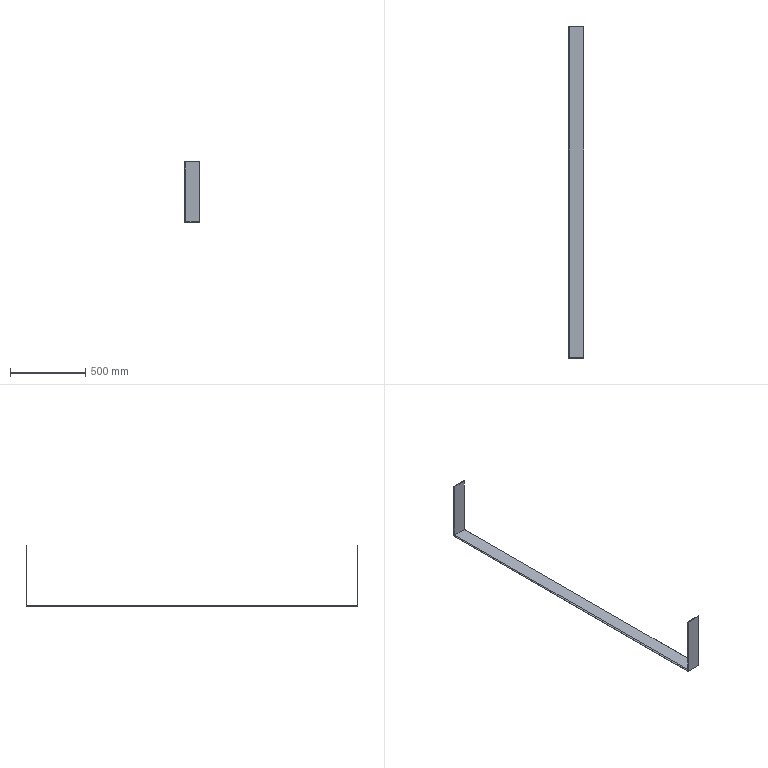Component | NX | FACA | 1 solid | 13 faces | box 100 x 2210 x 400 mm | volume 1452075 mm3 | plane 13
STEP:
#1=CARTESIAN_POINT('',(0.,0.,0.));
#2=DIRECTION('',(0.,0.,1.));
#3=DIRECTION('',(1.,0.,0.));
#4=AXIS2_PLACEMENT_3D('',#1,#2,#3);
#5=CARTESIAN_POINT('',(-710.,770.167,480.));
#6=VERTEX_POINT('',#5);
#7=CARTESIAN_POINT('',(-710.,770.167,80.));
#8=VERTEX_POINT('',#7);
#9=CARTESIAN_POINT('',(-710.,770.167,480.));
#10=DIRECTION('',(0.,0.,-1.));
#11=VECTOR('',#10,1.);
#12=LINE('',#9,#11);
#13=CARTESIAN_POINT('',(-810.,770.167,480.));
#14=DIRECTION('',(0.,-1.,0.));
#15=DIRECTION('',(0.,0.,1.));
#16=AXIS2_PLACEMENT_3D('',#13,#14,#15);
#17=PLANE('',#16);
#18=CARTESIAN_POINT('',(0.,-100.));
#19=DIRECTION('',(-1.,0.));
#20=VECTOR('',#19,1.);
#21=LINE('',#18,#20);
#22=(GEOMETRIC_REPRESENTATION_CONTEXT(2)PARAMETRIC_REPRESENTATION_CONTEXT()REPRESENTATION_CONTEXT('',''));
#23=DEFINITIONAL_REPRESENTATION('',(#21),#22);
#24=PCURVE('',#17,#23);
#25=CARTESIAN_POINT('',(-710.,770.167,80.));
#26=DIRECTION('',(-1.,0.,0.));
#27=DIRECTION('',(0.,0.,-1.));
#28=AXIS2_PLACEMENT_3D('',#25,#26,#27);
#29=PLANE('',#28);
#30=CARTESIAN_POINT('',(-400.,0.));
#31=DIRECTION('',(1.,0.));
#32=VECTOR('',#31,1.);
#33=LINE('',#30,#32);
#34=(GEOMETRIC_REPRESENTATION_CONTEXT(2)PARAMETRIC_REPRESENTATION_CONTEXT()REPRESENTATION_CONTEXT('',''));
#35=DEFINITIONAL_REPRESENTATION('',(#33),#34);
#36=PCURVE('',#29,#35);
#37=SURFACE_CURVE('',#12,(#24,#36),.PCURVE_S1.);
#38=EDGE_CURVE('',#6,#8,#37,.T.);
#39=ORIENTED_EDGE('',*,*,#38,.T.);
#40=CARTESIAN_POINT('',(-810.,770.167,80.));
#41=VERTEX_POINT('',#40);
#42=CARTESIAN_POINT('',(-810.,770.167,80.));
#43=DIRECTION('',(1.,0.,0.));
#44=VECTOR('',#43,1.);
#45=LINE('',#42,#44);
#46=CARTESIAN_POINT('',(-400.,0.));
#47=DIRECTION('',(0.,-1.));
#48=VECTOR('',#47,1.);
#49=LINE('',#46,#48);
#50=(GEOMETRIC_REPRESENTATION_CONTEXT(2)PARAMETRIC_REPRESENTATION_CONTEXT()REPRESENTATION_CONTEXT('',''));
#51=DEFINITIONAL_REPRESENTATION('',(#49),#50);
#52=PCURVE('',#17,#51);
#53=CARTESIAN_POINT('',(-810.,770.167,80.));
#54=DIRECTION('',(0.,0.,1.));
#55=DIRECTION('',(-1.,0.,0.));
#56=AXIS2_PLACEMENT_3D('',#53,#54,#55);
#57=PLANE('',#56);
#58=CARTESIAN_POINT('',(0.,0.));
#59=DIRECTION('',(-1.,0.));
#60=VECTOR('',#59,1.);
#61=LINE('',#58,#60);
#62=(GEOMETRIC_REPRESENTATION_CONTEXT(2)PARAMETRIC_REPRESENTATION_CONTEXT()REPRESENTATION_CONTEXT('',''));
#63=DEFINITIONAL_REPRESENTATION('',(#61),#62);
#64=PCURVE('',#57,#63);
#65=SURFACE_CURVE('',#45,(#52,#64),.PCURVE_S1.);
#66=EDGE_CURVE('',#41,#8,#65,.T.);
#67=ORIENTED_EDGE('',*,*,#66,.F.);
#68=CARTESIAN_POINT('',(-810.,770.167,480.));
#69=VERTEX_POINT('',#68);
#70=CARTESIAN_POINT('',(-810.,770.167,480.));
#71=DIRECTION('',(0.,0.,-1.));
#72=VECTOR('',#71,1.);
#73=LINE('',#70,#72);
#74=CARTESIAN_POINT('',(0.,0.));
#75=DIRECTION('',(-1.,0.));
#76=VECTOR('',#75,1.);
#77=LINE('',#74,#76);
#78=(GEOMETRIC_REPRESENTATION_CONTEXT(2)PARAMETRIC_REPRESENTATION_CONTEXT()REPRESENTATION_CONTEXT('',''));
#79=DEFINITIONAL_REPRESENTATION('',(#77),#78);
#80=PCURVE('',#17,#79);
#81=CARTESIAN_POINT('',(-810.,770.167,80.));
#82=DIRECTION('',(-1.,0.,0.));
#83=DIRECTION('',(0.,0.,-1.));
#84=AXIS2_PLACEMENT_3D('',#81,#82,#83);
#85=PLANE('',#84);
#86=CARTESIAN_POINT('',(-400.,0.));
#87=DIRECTION('',(1.,0.));
#88=VECTOR('',#87,1.);
#89=LINE('',#86,#88);
#90=(GEOMETRIC_REPRESENTATION_CONTEXT(2)PARAMETRIC_REPRESENTATION_CONTEXT()REPRESENTATION_CONTEXT('',''));
#91=DEFINITIONAL_REPRESENTATION('',(#89),#90);
#92=PCURVE('',#85,#91);
#93=SURFACE_CURVE('',#73,(#80,#92),.PCURVE_S1.);
#94=EDGE_CURVE('',#69,#41,#93,.T.);
#95=ORIENTED_EDGE('',*,*,#94,.F.);
#96=CARTESIAN_POINT('',(-810.,770.167,480.));
#97=DIRECTION('',(1.,0.,0.));
#98=VECTOR('',#97,1.);
#99=LINE('',#96,#98);
#100=CARTESIAN_POINT('',(0.,0.));
#101=DIRECTION('',(0.,-1.));
#102=VECTOR('',#101,1.);
#103=LINE('',#100,#102);
#104=(GEOMETRIC_REPRESENTATION_CONTEXT(2)PARAMETRIC_REPRESENTATION_CONTEXT()REPRESENTATION_CONTEXT('',''));
#105=DEFINITIONAL_REPRESENTATION('',(#103),#104);
#106=PCURVE('',#17,#105);
#107=CARTESIAN_POINT('',(-810.,765.167,480.));
#108=DIRECTION('',(0.,0.,-1.));
#109=DIRECTION('',(1.,0.,0.));
#110=AXIS2_PLACEMENT_3D('',#107,#108,#109);
#111=PLANE('',#110);
#112=CARTESIAN_POINT('',(0.,-5.));
#113=DIRECTION('',(1.,0.));
#114=VECTOR('',#113,1.);
#115=LINE('',#112,#114);
#116=(GEOMETRIC_REPRESENTATION_CONTEXT(2)PARAMETRIC_REPRESENTATION_CONTEXT()REPRESENTATION_CONTEXT('',''));
#117=DEFINITIONAL_REPRESENTATION('',(#115),#116);
#118=PCURVE('',#111,#117);
#119=SURFACE_CURVE('',#99,(#106,#118),.PCURVE_S1.);
#120=EDGE_CURVE('',#69,#6,#119,.T.);
#121=ORIENTED_EDGE('',*,*,#120,.T.);
#122=EDGE_LOOP('',(#39,#67,#95,#121));
#123=FACE_BOUND('',#122,.T.);
#124=ADVANCED_FACE('',(#123),#17,.F.);
#125=CARTESIAN_POINT('',(-710.,-1439.833,80.));
#126=VERTEX_POINT('',#125);
#127=CARTESIAN_POINT('',(-710.,770.167,80.));
#128=DIRECTION('',(0.,-1.,0.));
#129=VECTOR('',#128,1.);
#130=LINE('',#127,#129);
#131=CARTESIAN_POINT('',(-100.,0.));
#132=DIRECTION('',(0.,1.));
#133=VECTOR('',#132,1.);
#134=LINE('',#131,#133);
#135=(GEOMETRIC_REPRESENTATION_CONTEXT(2)PARAMETRIC_REPRESENTATION_CONTEXT()REPRESENTATION_CONTEXT('',''));
#136=DEFINITIONAL_REPRESENTATION('',(#134),#135);
#137=PCURVE('',#57,#136);
#138=CARTESIAN_POINT('',(0.,0.));
#139=DIRECTION('',(0.,1.));
#140=VECTOR('',#139,1.);
#141=LINE('',#138,#140);
#142=(GEOMETRIC_REPRESENTATION_CONTEXT(2)PARAMETRIC_REPRESENTATION_CONTEXT()REPRESENTATION_CONTEXT('',''));
#143=DEFINITIONAL_REPRESENTATION('',(#141),#142);
#144=PCURVE('',#29,#143);
#145=SURFACE_CURVE('',#130,(#137,#144),.PCURVE_S1.);
#146=EDGE_CURVE('',#8,#126,#145,.T.);
#147=ORIENTED_EDGE('',*,*,#146,.T.);
#148=CARTESIAN_POINT('',(-810.,-1439.833,80.));
#149=VERTEX_POINT('',#148);
#150=CARTESIAN_POINT('',(-810.,-1439.833,80.));
#151=DIRECTION('',(1.,0.,0.));
#152=VECTOR('',#151,1.);
#153=LINE('',#150,#152);
#154=CARTESIAN_POINT('',(0.,2210.));
#155=DIRECTION('',(-1.,0.));
#156=VECTOR('',#155,1.);
#157=LINE('',#154,#156);
#158=(GEOMETRIC_REPRESENTATION_CONTEXT(2)PARAMETRIC_REPRESENTATION_CONTEXT()REPRESENTATION_CONTEXT('',''));
#159=DEFINITIONAL_REPRESENTATION('',(#157),#158);
#160=PCURVE('',#57,#159);
#161=CARTESIAN_POINT('',(-810.,-1439.833,80.));
#162=DIRECTION('',(0.,1.,0.));
#163=DIRECTION('',(0.,0.,-1.));
#164=AXIS2_PLACEMENT_3D('',#161,#162,#163);
#165=PLANE('',#164);
#166=CARTESIAN_POINT('',(0.,0.));
#167=DIRECTION('',(0.,-1.));
#168=VECTOR('',#167,1.);
#169=LINE('',#166,#168);
#170=(GEOMETRIC_REPRESENTATION_CONTEXT(2)PARAMETRIC_REPRESENTATION_CONTEXT()REPRESENTATION_CONTEXT('',''));
#171=DEFINITIONAL_REPRESENTATION('',(#169),#170);
#172=PCURVE('',#165,#171);
#173=SURFACE_CURVE('',#153,(#160,#172),.PCURVE_S1.);
#174=EDGE_CURVE('',#149,#126,#173,.T.);
#175=ORIENTED_EDGE('',*,*,#174,.F.);
#176=CARTESIAN_POINT('',(-810.,770.167,80.));
#177=DIRECTION('',(0.,-1.,0.));
#178=VECTOR('',#177,1.);
#179=LINE('',#176,#178);
#180=CARTESIAN_POINT('',(0.,0.));
#181=DIRECTION('',(0.,1.));
#182=VECTOR('',#181,1.);
#183=LINE('',#180,#182);
#184=(GEOMETRIC_REPRESENTATION_CONTEXT(2)PARAMETRIC_REPRESENTATION_CONTEXT()REPRESENTATION_CONTEXT('',''));
#185=DEFINITIONAL_REPRESENTATION('',(#183),#184);
#186=PCURVE('',#57,#185);
#187=CARTESIAN_POINT('',(0.,0.));
#188=DIRECTION('',(0.,1.));
#189=VECTOR('',#188,1.);
#190=LINE('',#187,#189);
#191=(GEOMETRIC_REPRESENTATION_CONTEXT(2)PARAMETRIC_REPRESENTATION_CONTEXT()REPRESENTATION_CONTEXT('',''));
#192=DEFINITIONAL_REPRESENTATION('',(#190),#191);
#193=PCURVE('',#85,#192);
#194=SURFACE_CURVE('',#179,(#186,#193),.PCURVE_S1.);
#195=EDGE_CURVE('',#41,#149,#194,.T.);
#196=ORIENTED_EDGE('',*,*,#195,.F.);
#197=ORIENTED_EDGE('',*,*,#66,.T.);
#198=EDGE_LOOP('',(#147,#175,#196,#197));
#199=FACE_BOUND('',#198,.T.);
#200=ADVANCED_FACE('',(#199),#57,.F.);
#201=CARTESIAN_POINT('',(-710.,-1439.833,480.));
#202=VERTEX_POINT('',#201);
#203=CARTESIAN_POINT('',(-710.,-1439.833,80.));
#204=DIRECTION('',(0.,0.,1.));
#205=VECTOR('',#204,1.);
#206=LINE('',#203,#205);
#207=CARTESIAN_POINT('',(0.,-100.));
#208=DIRECTION('',(-1.,0.));
#209=VECTOR('',#208,1.);
#210=LINE('',#207,#209);
#211=(GEOMETRIC_REPRESENTATION_CONTEXT(2)PARAMETRIC_REPRESENTATION_CONTEXT()REPRESENTATION_CONTEXT('',''));
#212=DEFINITIONAL_REPRESENTATION('',(#210),#211);
#213=PCURVE('',#165,#212);
#214=CARTESIAN_POINT('',(0.,2210.));
#215=DIRECTION('',(-1.,0.));
#216=VECTOR('',#215,1.);
#217=LINE('',#214,#216);
#218=(GEOMETRIC_REPRESENTATION_CONTEXT(2)PARAMETRIC_REPRESENTATION_CONTEXT()REPRESENTATION_CONTEXT('',''));
#219=DEFINITIONAL_REPRESENTATION('',(#217),#218);
#220=PCURVE('',#29,#219);
#221=SURFACE_CURVE('',#206,(#213,#220),.PCURVE_S1.);
#222=EDGE_CURVE('',#126,#202,#221,.T.);
#223=ORIENTED_EDGE('',*,*,#222,.T.);
#224=CARTESIAN_POINT('',(-810.,-1439.833,480.));
#225=VERTEX_POINT('',#224);
#226=CARTESIAN_POINT('',(-810.,-1439.833,480.));
#227=DIRECTION('',(1.,0.,0.));
#228=VECTOR('',#227,1.);
#229=LINE('',#226,#228);
#230=CARTESIAN_POINT('',(-400.,0.));
#231=DIRECTION('',(0.,-1.));
#232=VECTOR('',#231,1.);
#233=LINE('',#230,#232);
#234=(GEOMETRIC_REPRESENTATION_CONTEXT(2)PARAMETRIC_REPRESENTATION_CONTEXT()REPRESENTATION_CONTEXT('',''));
#235=DEFINITIONAL_REPRESENTATION('',(#233),#234);
#236=PCURVE('',#165,#235);
#237=CARTESIAN_POINT('',(-810.,-1439.833,480.));
#238=DIRECTION('',(0.,0.,-1.));
#239=DIRECTION('',(1.,0.,0.));
#240=AXIS2_PLACEMENT_3D('',#237,#238,#239);
#241=PLANE('',#240);
#242=CARTESIAN_POINT('',(0.,0.));
#243=DIRECTION('',(1.,0.));
#244=VECTOR('',#243,1.);
#245=LINE('',#242,#244);
#246=(GEOMETRIC_REPRESENTATION_CONTEXT(2)PARAMETRIC_REPRESENTATION_CONTEXT()REPRESENTATION_CONTEXT('',''));
#247=DEFINITIONAL_REPRESENTATION('',(#245),#246);
#248=PCURVE('',#241,#247);
#249=SURFACE_CURVE('',#229,(#236,#248),.PCURVE_S1.);
#250=EDGE_CURVE('',#225,#202,#249,.T.);
#251=ORIENTED_EDGE('',*,*,#250,.F.);
#252=CARTESIAN_POINT('',(-810.,-1439.833,80.));
#253=DIRECTION('',(0.,0.,1.));
#254=VECTOR('',#253,1.);
#255=LINE('',#252,#254);
#256=CARTESIAN_POINT('',(0.,0.));
#257=DIRECTION('',(-1.,0.));
#258=VECTOR('',#257,1.);
#259=LINE('',#256,#258);
#260=(GEOMETRIC_REPRESENTATION_CONTEXT(2)PARAMETRIC_REPRESENTATION_CONTEXT()REPRESENTATION_CONTEXT('',''));
#261=DEFINITIONAL_REPRESENTATION('',(#259),#260);
#262=PCURVE('',#165,#261);
#263=CARTESIAN_POINT('',(0.,2210.));
#264=DIRECTION('',(-1.,0.));
#265=VECTOR('',#264,1.);
#266=LINE('',#263,#265);
#267=(GEOMETRIC_REPRESENTATION_CONTEXT(2)PARAMETRIC_REPRESENTATION_CONTEXT()REPRESENTATION_CONTEXT('',''));
#268=DEFINITIONAL_REPRESENTATION('',(#266),#267);
#269=PCURVE('',#85,#268);
#270=SURFACE_CURVE('',#255,(#262,#269),.PCURVE_S1.);
#271=EDGE_CURVE('',#149,#225,#270,.T.);
#272=ORIENTED_EDGE('',*,*,#271,.F.);
#273=ORIENTED_EDGE('',*,*,#174,.T.);
#274=EDGE_LOOP('',(#223,#251,#272,#273));
#275=FACE_BOUND('',#274,.T.);
#276=ADVANCED_FACE('',(#275),#165,.F.);
#277=CARTESIAN_POINT('',(-802.,-1434.833,480.));
#278=VERTEX_POINT('',#277);
#279=CARTESIAN_POINT('',(-710.,-1434.833,480.));
#280=VERTEX_POINT('',#279);
#281=CARTESIAN_POINT('',(-810.,-1434.833,480.));
#282=DIRECTION('',(1.,0.,0.));
#283=VECTOR('',#282,1.);
#284=LINE('',#281,#283);
#285=CARTESIAN_POINT('',(0.,-5.));
#286=DIRECTION('',(1.,0.));
#287=VECTOR('',#286,1.);
#288=LINE('',#285,#287);
#289=(GEOMETRIC_REPRESENTATION_CONTEXT(2)PARAMETRIC_REPRESENTATION_CONTEXT()REPRESENTATION_CONTEXT('',''));
#290=DEFINITIONAL_REPRESENTATION('',(#288),#289);
#291=PCURVE('',#241,#290);
#292=CARTESIAN_POINT('',(-810.,-1434.833,480.));
#293=DIRECTION('',(0.,-1.,0.));
#294=DIRECTION('',(0.,0.,1.));
#295=AXIS2_PLACEMENT_3D('',#292,#293,#294);
#296=PLANE('',#295);
#297=CARTESIAN_POINT('',(0.,0.));
#298=DIRECTION('',(0.,-1.));
#299=VECTOR('',#298,1.);
#300=LINE('',#297,#299);
#301=(GEOMETRIC_REPRESENTATION_CONTEXT(2)PARAMETRIC_REPRESENTATION_CONTEXT()REPRESENTATION_CONTEXT('',''));
#302=DEFINITIONAL_REPRESENTATION('',(#300),#301);
#303=PCURVE('',#296,#302);
#304=SURFACE_CURVE('',#284,(#291,#303),.PCURVE_S1.);
#305=EDGE_CURVE('',#278,#280,#304,.T.);
#306=ORIENTED_EDGE('',*,*,#305,.F.);
#307=CARTESIAN_POINT('',(-810.,-1438.833,480.));
#308=VERTEX_POINT('',#307);
#309=CARTESIAN_POINT('',(-810.,-1438.833,480.));
#310=DIRECTION('',(-0.8944,-0.4472,0.));
#311=VECTOR('',#310,1.);
#312=LINE('',#309,#311);
#313=CARTESIAN_POINT('',(0.,-1.));
#314=DIRECTION('',(-0.8944,0.4472));
#315=VECTOR('',#314,1.);
#316=LINE('',#313,#315);
#317=(GEOMETRIC_REPRESENTATION_CONTEXT(2)PARAMETRIC_REPRESENTATION_CONTEXT()REPRESENTATION_CONTEXT('',''));
#318=DEFINITIONAL_REPRESENTATION('',(#316),#317);
#319=PCURVE('',#241,#318);
#320=CARTESIAN_POINT('',(-810.,-1438.833,80.));
#321=DIRECTION('',(-0.4472,0.8944,0.));
#322=DIRECTION('',(0.,0.,1.));
#323=AXIS2_PLACEMENT_3D('',#320,#321,#322);
#324=PLANE('',#323);
#325=CARTESIAN_POINT('',(400.,0.));
#326=DIRECTION('',(0.,-1.));
#327=VECTOR('',#326,1.);
#328=LINE('',#325,#327);
#329=(GEOMETRIC_REPRESENTATION_CONTEXT(2)PARAMETRIC_REPRESENTATION_CONTEXT()REPRESENTATION_CONTEXT('',''));
#330=DEFINITIONAL_REPRESENTATION('',(#328),#329);
#331=PCURVE('',#324,#330);
#332=SURFACE_CURVE('',#312,(#319,#331),.PCURVE_S1.);
#333=EDGE_CURVE('',#278,#308,#332,.T.);
#334=ORIENTED_EDGE('',*,*,#333,.T.);
#335=CARTESIAN_POINT('',(-810.,-1439.833,480.));
#336=DIRECTION('',(0.,1.,0.));
#337=VECTOR('',#336,1.);
#338=LINE('',#335,#337);
#339=CARTESIAN_POINT('',(0.,0.));
#340=DIRECTION('',(0.,-1.));
#341=VECTOR('',#340,1.);
#342=LINE('',#339,#341);
#343=(GEOMETRIC_REPRESENTATION_CONTEXT(2)PARAMETRIC_REPRESENTATION_CONTEXT()REPRESENTATION_CONTEXT('',''));
#344=DEFINITIONAL_REPRESENTATION('',(#342),#343);
#345=PCURVE('',#241,#344);
#346=CARTESIAN_POINT('',(-400.,2210.));
#347=DIRECTION('',(0.,-1.));
#348=VECTOR('',#347,1.);
#349=LINE('',#346,#348);
#350=(GEOMETRIC_REPRESENTATION_CONTEXT(2)PARAMETRIC_REPRESENTATION_CONTEXT()REPRESENTATION_CONTEXT('',''));
#351=DEFINITIONAL_REPRESENTATION('',(#349),#350);
#352=PCURVE('',#85,#351);
#353=SURFACE_CURVE('',#338,(#345,#352),.PCURVE_S1.);
#354=EDGE_CURVE('',#225,#308,#353,.T.);
#355=ORIENTED_EDGE('',*,*,#354,.F.);
#356=ORIENTED_EDGE('',*,*,#250,.T.);
#357=CARTESIAN_POINT('',(-710.,-1439.833,480.));
#358=DIRECTION('',(0.,1.,0.));
#359=VECTOR('',#358,1.);
#360=LINE('',#357,#359);
#361=CARTESIAN_POINT('',(100.,0.));
#362=DIRECTION('',(0.,-1.));
#363=VECTOR('',#362,1.);
#364=LINE('',#361,#363);
#365=(GEOMETRIC_REPRESENTATION_CONTEXT(2)PARAMETRIC_REPRESENTATION_CONTEXT()REPRESENTATION_CONTEXT('',''));
#366=DEFINITIONAL_REPRESENTATION('',(#364),#365);
#367=PCURVE('',#241,#366);
#368=CARTESIAN_POINT('',(-400.,2210.));
#369=DIRECTION('',(0.,-1.));
#370=VECTOR('',#369,1.);
#371=LINE('',#368,#370);
#372=(GEOMETRIC_REPRESENTATION_CONTEXT(2)PARAMETRIC_REPRESENTATION_CONTEXT()REPRESENTATION_CONTEXT('',''));
#373=DEFINITIONAL_REPRESENTATION('',(#371),#372);
#374=PCURVE('',#29,#373);
#375=SURFACE_CURVE('',#360,(#367,#374),.PCURVE_S1.);
#376=EDGE_CURVE('',#202,#280,#375,.T.);
#377=ORIENTED_EDGE('',*,*,#376,.T.);
#378=EDGE_LOOP('',(#306,#334,#355,#356,#377));
#379=FACE_BOUND('',#378,.T.);
#380=ADVANCED_FACE('',(#379),#241,.F.);
#381=CARTESIAN_POINT('',(-802.,-1434.833,85.));
#382=VERTEX_POINT('',#381);
#383=CARTESIAN_POINT('',(-710.,-1434.833,85.));
#384=VERTEX_POINT('',#383);
#385=CARTESIAN_POINT('',(-810.,-1434.833,85.));
#386=DIRECTION('',(1.,0.,0.));
#387=VECTOR('',#386,1.);
#388=LINE('',#385,#387);
#389=CARTESIAN_POINT('',(-395.,0.));
#390=DIRECTION('',(0.,-1.));
#391=VECTOR('',#390,1.);
#392=LINE('',#389,#391);
#393=(GEOMETRIC_REPRESENTATION_CONTEXT(2)PARAMETRIC_REPRESENTATION_CONTEXT()REPRESENTATION_CONTEXT('',''));
#394=DEFINITIONAL_REPRESENTATION('',(#392),#393);
#395=PCURVE('',#296,#394);
#396=CARTESIAN_POINT('',(-810.,-1434.833,85.));
#397=DIRECTION('',(0.,0.,-1.));
#398=DIRECTION('',(1.,0.,0.));
#399=AXIS2_PLACEMENT_3D('',#396,#397,#398);
#400=PLANE('',#399);
#401=CARTESIAN_POINT('',(0.,0.));
#402=DIRECTION('',(1.,0.));
#403=VECTOR('',#402,1.);
#404=LINE('',#401,#403);
#405=(GEOMETRIC_REPRESENTATION_CONTEXT(2)PARAMETRIC_REPRESENTATION_CONTEXT()REPRESENTATION_CONTEXT('',''));
#406=DEFINITIONAL_REPRESENTATION('',(#404),#405);
#407=PCURVE('',#400,#406);
#408=SURFACE_CURVE('',#388,(#395,#407),.PCURVE_S1.);
#409=EDGE_CURVE('',#382,#384,#408,.T.);
#410=ORIENTED_EDGE('',*,*,#409,.F.);
#411=CARTESIAN_POINT('',(-802.,-1434.833,480.));
#412=DIRECTION('',(0.,0.,1.));
#413=VECTOR('',#412,1.);
#414=LINE('',#411,#413);
#415=CARTESIAN_POINT('',(0.,-8.));
#416=DIRECTION('',(1.,0.));
#417=VECTOR('',#416,1.);
#418=LINE('',#415,#417);
#419=(GEOMETRIC_REPRESENTATION_CONTEXT(2)PARAMETRIC_REPRESENTATION_CONTEXT()REPRESENTATION_CONTEXT('',''));
#420=DEFINITIONAL_REPRESENTATION('',(#418),#419);
#421=PCURVE('',#296,#420);
#422=CARTESIAN_POINT('',(400.,8.944));
#423=DIRECTION('',(1.,0.));
#424=VECTOR('',#423,1.);
#425=LINE('',#422,#424);
#426=(GEOMETRIC_REPRESENTATION_CONTEXT(2)PARAMETRIC_REPRESENTATION_CONTEXT()REPRESENTATION_CONTEXT('',''));
#427=DEFINITIONAL_REPRESENTATION('',(#425),#426);
#428=PCURVE('',#324,#427);
#429=SURFACE_CURVE('',#414,(#421,#428),.PCURVE_S1.);
#430=EDGE_CURVE('',#382,#278,#429,.T.);
#431=ORIENTED_EDGE('',*,*,#430,.T.);
#432=ORIENTED_EDGE('',*,*,#305,.T.);
#433=CARTESIAN_POINT('',(-710.,-1434.833,480.));
#434=DIRECTION('',(0.,0.,-1.));
#435=VECTOR('',#434,1.);
#436=LINE('',#433,#435);
#437=CARTESIAN_POINT('',(0.,-100.));
#438=DIRECTION('',(-1.,0.));
#439=VECTOR('',#438,1.);
#440=LINE('',#437,#439);
#441=(GEOMETRIC_REPRESENTATION_CONTEXT(2)PARAMETRIC_REPRESENTATION_CONTEXT()REPRESENTATION_CONTEXT('',''));
#442=DEFINITIONAL_REPRESENTATION('',(#440),#441);
#443=PCURVE('',#296,#442);
#444=CARTESIAN_POINT('',(-400.,2205.));
#445=DIRECTION('',(1.,0.));
#446=VECTOR('',#445,1.);
#447=LINE('',#444,#446);
#448=(GEOMETRIC_REPRESENTATION_CONTEXT(2)PARAMETRIC_REPRESENTATION_CONTEXT()REPRESENTATION_CONTEXT('',''));
#449=DEFINITIONAL_REPRESENTATION('',(#447),#448);
#450=PCURVE('',#29,#449);
#451=SURFACE_CURVE('',#436,(#443,#450),.PCURVE_S1.);
#452=EDGE_CURVE('',#280,#384,#451,.T.);
#453=ORIENTED_EDGE('',*,*,#452,.T.);
#454=EDGE_LOOP('',(#410,#431,#432,#453));
#455=FACE_BOUND('',#454,.T.);
#456=ADVANCED_FACE('',(#455),#296,.F.);
#457=CARTESIAN_POINT('',(-802.,765.167,85.));
#458=VERTEX_POINT('',#457);
#459=CARTESIAN_POINT('',(-710.,765.167,85.));
#460=VERTEX_POINT('',#459);
#461=CARTESIAN_POINT('',(-810.,765.167,85.));
#462=DIRECTION('',(1.,0.,0.));
#463=VECTOR('',#462,1.);
#464=LINE('',#461,#463);
#465=CARTESIAN_POINT('',(0.,-2200.));
#466=DIRECTION('',(1.,0.));
#467=VECTOR('',#466,1.);
#468=LINE('',#465,#467);
#469=(GEOMETRIC_REPRESENTATION_CONTEXT(2)PARAMETRIC_REPRESENTATION_CONTEXT()REPRESENTATION_CONTEXT('',''));
#470=DEFINITIONAL_REPRESENTATION('',(#468),#469);
#471=PCURVE('',#400,#470);
#472=CARTESIAN_POINT('',(-810.,765.167,85.));
#473=DIRECTION('',(0.,1.,0.));
#474=DIRECTION('',(0.,0.,-1.));
#475=AXIS2_PLACEMENT_3D('',#472,#473,#474);
#476=PLANE('',#475);
#477=CARTESIAN_POINT('',(0.,0.));
#478=DIRECTION('',(0.,-1.));
#479=VECTOR('',#478,1.);
#480=LINE('',#477,#479);
#481=(GEOMETRIC_REPRESENTATION_CONTEXT(2)PARAMETRIC_REPRESENTATION_CONTEXT()REPRESENTATION_CONTEXT('',''));
#482=DEFINITIONAL_REPRESENTATION('',(#480),#481);
#483=PCURVE('',#476,#482);
#484=SURFACE_CURVE('',#464,(#471,#483),.PCURVE_S1.);
#485=EDGE_CURVE('',#458,#460,#484,.T.);
#486=ORIENTED_EDGE('',*,*,#485,.F.);
#487=CARTESIAN_POINT('',(-802.,-1434.833,85.));
#488=DIRECTION('',(0.,-1.,0.));
#489=VECTOR('',#488,1.);
#490=LINE('',#487,#489);
#491=CARTESIAN_POINT('',(8.,0.));
#492=DIRECTION('',(0.,1.));
#493=VECTOR('',#492,1.);
#494=LINE('',#491,#493);
#495=(GEOMETRIC_REPRESENTATION_CONTEXT(2)PARAMETRIC_REPRESENTATION_CONTEXT()REPRESENTATION_CONTEXT('',''));
#496=DEFINITIONAL_REPRESENTATION('',(#494),#495);
#497=PCURVE('',#400,#496);
#498=CARTESIAN_POINT('',(-810.,770.167,81.));
#499=DIRECTION('',(-0.4472,0.,0.8944));
#500=DIRECTION('',(0.,-1.,0.));
#501=AXIS2_PLACEMENT_3D('',#498,#499,#500);
#502=PLANE('',#501);
#503=CARTESIAN_POINT('',(2205.,8.944));
#504=DIRECTION('',(1.,0.));
#505=VECTOR('',#504,1.);
#506=LINE('',#503,#505);
#507=(GEOMETRIC_REPRESENTATION_CONTEXT(2)PARAMETRIC_REPRESENTATION_CONTEXT()REPRESENTATION_CONTEXT('',''));
#508=DEFINITIONAL_REPRESENTATION('',(#506),#507);
#509=PCURVE('',#502,#508);
#510=SURFACE_CURVE('',#490,(#497,#509),.PCURVE_S1.);
#511=EDGE_CURVE('',#458,#382,#510,.T.);
#512=ORIENTED_EDGE('',*,*,#511,.T.);
#513=ORIENTED_EDGE('',*,*,#409,.T.);
#514=CARTESIAN_POINT('',(-710.,-1434.833,85.));
#515=DIRECTION('',(0.,1.,0.));
#516=VECTOR('',#515,1.);
#517=LINE('',#514,#516);
#518=CARTESIAN_POINT('',(100.,0.));
#519=DIRECTION('',(0.,-1.));
#520=VECTOR('',#519,1.);
#521=LINE('',#518,#520);
#522=(GEOMETRIC_REPRESENTATION_CONTEXT(2)PARAMETRIC_REPRESENTATION_CONTEXT()REPRESENTATION_CONTEXT('',''));
#523=DEFINITIONAL_REPRESENTATION('',(#521),#522);
#524=PCURVE('',#400,#523);
#525=CARTESIAN_POINT('',(-5.,2205.));
#526=DIRECTION('',(0.,-1.));
#527=VECTOR('',#526,1.);
#528=LINE('',#525,#527);
#529=(GEOMETRIC_REPRESENTATION_CONTEXT(2)PARAMETRIC_REPRESENTATION_CONTEXT()REPRESENTATION_CONTEXT('',''));
#530=DEFINITIONAL_REPRESENTATION('',(#528),#529);
#531=PCURVE('',#29,#530);
#532=SURFACE_CURVE('',#517,(#524,#531),.PCURVE_S1.);
#533=EDGE_CURVE('',#384,#460,#532,.T.);
#534=ORIENTED_EDGE('',*,*,#533,.T.);
#535=EDGE_LOOP('',(#486,#512,#513,#534));
#536=FACE_BOUND('',#535,.T.);
#537=ADVANCED_FACE('',(#536),#400,.F.);
#538=CARTESIAN_POINT('',(-802.,765.167,480.));
#539=VERTEX_POINT('',#538);
#540=CARTESIAN_POINT('',(-710.,765.167,480.));
#541=VERTEX_POINT('',#540);
#542=CARTESIAN_POINT('',(-810.,765.167,480.));
#543=DIRECTION('',(1.,0.,0.));
#544=VECTOR('',#543,1.);
#545=LINE('',#542,#544);
#546=CARTESIAN_POINT('',(-395.,0.));
#547=DIRECTION('',(0.,-1.));
#548=VECTOR('',#547,1.);
#549=LINE('',#546,#548);
#550=(GEOMETRIC_REPRESENTATION_CONTEXT(2)PARAMETRIC_REPRESENTATION_CONTEXT()REPRESENTATION_CONTEXT('',''));
#551=DEFINITIONAL_REPRESENTATION('',(#549),#550);
#552=PCURVE('',#476,#551);
#553=CARTESIAN_POINT('',(0.,0.));
#554=DIRECTION('',(1.,0.));
#555=VECTOR('',#554,1.);
#556=LINE('',#553,#555);
#557=(GEOMETRIC_REPRESENTATION_CONTEXT(2)PARAMETRIC_REPRESENTATION_CONTEXT()REPRESENTATION_CONTEXT('',''));
#558=DEFINITIONAL_REPRESENTATION('',(#556),#557);
#559=PCURVE('',#111,#558);
#560=SURFACE_CURVE('',#545,(#552,#559),.PCURVE_S1.);
#561=EDGE_CURVE('',#539,#541,#560,.T.);
#562=ORIENTED_EDGE('',*,*,#561,.F.);
#563=CARTESIAN_POINT('',(-802.,765.167,85.));
#564=DIRECTION('',(0.,0.,-1.));
#565=VECTOR('',#564,1.);
#566=LINE('',#563,#565);
#567=CARTESIAN_POINT('',(0.,-8.));
#568=DIRECTION('',(1.,0.));
#569=VECTOR('',#568,1.);
#570=LINE('',#567,#569);
#571=(GEOMETRIC_REPRESENTATION_CONTEXT(2)PARAMETRIC_REPRESENTATION_CONTEXT()REPRESENTATION_CONTEXT('',''));
#572=DEFINITIONAL_REPRESENTATION('',(#570),#571);
#573=PCURVE('',#476,#572);
#574=CARTESIAN_POINT('',(-810.,769.167,80.));
#575=DIRECTION('',(-0.4472,-0.8944,0.));
#576=DIRECTION('',(0.,0.,-1.));
#577=AXIS2_PLACEMENT_3D('',#574,#575,#576);
#578=PLANE('',#577);
#579=CARTESIAN_POINT('',(-5.,8.944));
#580=DIRECTION('',(1.,0.));
#581=VECTOR('',#580,1.);
#582=LINE('',#579,#581);
#583=(GEOMETRIC_REPRESENTATION_CONTEXT(2)PARAMETRIC_REPRESENTATION_CONTEXT()REPRESENTATION_CONTEXT('',''));
#584=DEFINITIONAL_REPRESENTATION('',(#582),#583);
#585=PCURVE('',#578,#584);
#586=SURFACE_CURVE('',#566,(#573,#585),.PCURVE_S1.);
#587=EDGE_CURVE('',#539,#458,#586,.T.);
#588=ORIENTED_EDGE('',*,*,#587,.T.);
#589=ORIENTED_EDGE('',*,*,#485,.T.);
#590=CARTESIAN_POINT('',(-710.,765.167,85.));
#591=DIRECTION('',(0.,0.,1.));
#592=VECTOR('',#591,1.);
#593=LINE('',#590,#592);
#594=CARTESIAN_POINT('',(0.,-100.));
#595=DIRECTION('',(-1.,0.));
#596=VECTOR('',#595,1.);
#597=LINE('',#594,#596);
#598=(GEOMETRIC_REPRESENTATION_CONTEXT(2)PARAMETRIC_REPRESENTATION_CONTEXT()REPRESENTATION_CONTEXT('',''));
#599=DEFINITIONAL_REPRESENTATION('',(#597),#598);
#600=PCURVE('',#476,#599);
#601=CARTESIAN_POINT('',(-5.,5.));
#602=DIRECTION('',(-1.,0.));
#603=VECTOR('',#602,1.);
#604=LINE('',#601,#603);
#605=(GEOMETRIC_REPRESENTATION_CONTEXT(2)PARAMETRIC_REPRESENTATION_CONTEXT()REPRESENTATION_CONTEXT('',''));
#606=DEFINITIONAL_REPRESENTATION('',(#604),#605);
#607=PCURVE('',#29,#606);
#608=SURFACE_CURVE('',#593,(#600,#607),.PCURVE_S1.);
#609=EDGE_CURVE('',#460,#541,#608,.T.);
#610=ORIENTED_EDGE('',*,*,#609,.T.);
#611=EDGE_LOOP('',(#562,#588,#589,#610));
#612=FACE_BOUND('',#611,.T.);
#613=ADVANCED_FACE('',(#612),#476,.F.);
#614=CARTESIAN_POINT('',(-810.,769.167,480.));
#615=VERTEX_POINT('',#614);
#616=CARTESIAN_POINT('',(-810.,765.167,480.));
#617=DIRECTION('',(0.,1.,0.));
#618=VECTOR('',#617,1.);
#619=LINE('',#616,#618);
#620=CARTESIAN_POINT('',(0.,0.));
#621=DIRECTION('',(0.,-1.));
#622=VECTOR('',#621,1.);
#623=LINE('',#620,#622);
#624=(GEOMETRIC_REPRESENTATION_CONTEXT(2)PARAMETRIC_REPRESENTATION_CONTEXT()REPRESENTATION_CONTEXT('',''));
#625=DEFINITIONAL_REPRESENTATION('',(#623),#624);
#626=PCURVE('',#111,#625);
#627=CARTESIAN_POINT('',(-400.,5.));
#628=DIRECTION('',(0.,-1.));
#629=VECTOR('',#628,1.);
#630=LINE('',#627,#629);
#631=(GEOMETRIC_REPRESENTATION_CONTEXT(2)PARAMETRIC_REPRESENTATION_CONTEXT()REPRESENTATION_CONTEXT('',''));
#632=DEFINITIONAL_REPRESENTATION('',(#630),#631);
#633=PCURVE('',#85,#632);
#634=SURFACE_CURVE('',#619,(#626,#633),.PCURVE_S1.);
#635=EDGE_CURVE('',#615,#69,#634,.T.);
#636=ORIENTED_EDGE('',*,*,#635,.F.);
#637=CARTESIAN_POINT('',(-810.,769.167,480.));
#638=DIRECTION('',(0.8944,-0.4472,0.));
#639=VECTOR('',#638,1.);
#640=LINE('',#637,#639);
#641=CARTESIAN_POINT('',(0.,-4.));
#642=DIRECTION('',(0.8944,0.4472));
#643=VECTOR('',#642,1.);
#644=LINE('',#641,#643);
#645=(GEOMETRIC_REPRESENTATION_CONTEXT(2)PARAMETRIC_REPRESENTATION_CONTEXT()REPRESENTATION_CONTEXT('',''));
#646=DEFINITIONAL_REPRESENTATION('',(#644),#645);
#647=PCURVE('',#111,#646);
#648=CARTESIAN_POINT('',(-400.,0.));
#649=DIRECTION('',(0.,1.));
#650=VECTOR('',#649,1.);
#651=LINE('',#648,#650);
#652=(GEOMETRIC_REPRESENTATION_CONTEXT(2)PARAMETRIC_REPRESENTATION_CONTEXT()REPRESENTATION_CONTEXT('',''));
#653=DEFINITIONAL_REPRESENTATION('',(#651),#652);
#654=PCURVE('',#578,#653);
#655=SURFACE_CURVE('',#640,(#647,#654),.PCURVE_S1.);
#656=EDGE_CURVE('',#615,#539,#655,.T.);
#657=ORIENTED_EDGE('',*,*,#656,.T.);
#658=ORIENTED_EDGE('',*,*,#561,.T.);
#659=CARTESIAN_POINT('',(-710.,765.167,480.));
#660=DIRECTION('',(0.,1.,0.));
#661=VECTOR('',#660,1.);
#662=LINE('',#659,#661);
#663=CARTESIAN_POINT('',(100.,0.));
#664=DIRECTION('',(0.,-1.));
#665=VECTOR('',#664,1.);
#666=LINE('',#663,#665);
#667=(GEOMETRIC_REPRESENTATION_CONTEXT(2)PARAMETRIC_REPRESENTATION_CONTEXT()REPRESENTATION_CONTEXT('',''));
#668=DEFINITIONAL_REPRESENTATION('',(#666),#667);
#669=PCURVE('',#111,#668);
#670=CARTESIAN_POINT('',(-400.,5.));
#671=DIRECTION('',(0.,-1.));
#672=VECTOR('',#671,1.);
#673=LINE('',#670,#672);
#674=(GEOMETRIC_REPRESENTATION_CONTEXT(2)PARAMETRIC_REPRESENTATION_CONTEXT()REPRESENTATION_CONTEXT('',''));
#675=DEFINITIONAL_REPRESENTATION('',(#673),#674);
#676=PCURVE('',#29,#675);
#677=SURFACE_CURVE('',#662,(#669,#676),.PCURVE_S1.);
#678=EDGE_CURVE('',#541,#6,#677,.T.);
#679=ORIENTED_EDGE('',*,*,#678,.T.);
#680=ORIENTED_EDGE('',*,*,#120,.F.);
#681=EDGE_LOOP('',(#636,#657,#658,#679,#680));
#682=FACE_BOUND('',#681,.T.);
#683=ADVANCED_FACE('',(#682),#111,.F.);
#684=ORIENTED_EDGE('',*,*,#354,.T.);
#685=CARTESIAN_POINT('',(-810.,-1438.833,81.));
#686=VERTEX_POINT('',#685);
#687=CARTESIAN_POINT('',(-810.,-1438.833,85.));
#688=DIRECTION('',(0.,0.,-1.));
#689=VECTOR('',#688,1.);
#690=LINE('',#687,#689);
#691=CARTESIAN_POINT('',(-5.,2209.));
#692=DIRECTION('',(1.,0.));
#693=VECTOR('',#692,1.);
#694=LINE('',#691,#693);
#695=(GEOMETRIC_REPRESENTATION_CONTEXT(2)PARAMETRIC_REPRESENTATION_CONTEXT()REPRESENTATION_CONTEXT('',''));
#696=DEFINITIONAL_REPRESENTATION('',(#694),#695);
#697=PCURVE('',#85,#696);
#698=CARTESIAN_POINT('',(5.,0.));
#699=DIRECTION('',(-1.,0.));
#700=VECTOR('',#699,1.);
#701=LINE('',#698,#700);
#702=(GEOMETRIC_REPRESENTATION_CONTEXT(2)PARAMETRIC_REPRESENTATION_CONTEXT()REPRESENTATION_CONTEXT('',''));
#703=DEFINITIONAL_REPRESENTATION('',(#701),#702);
#704=PCURVE('',#324,#703);
#705=SURFACE_CURVE('',#690,(#697,#704),.PCURVE_S1.);
#706=EDGE_CURVE('',#308,#686,#705,.T.);
#707=ORIENTED_EDGE('',*,*,#706,.T.);
#708=CARTESIAN_POINT('',(-810.,769.167,81.));
#709=VERTEX_POINT('',#708);
#710=CARTESIAN_POINT('',(-810.,765.167,81.));
#711=DIRECTION('',(0.,1.,0.));
#712=VECTOR('',#711,1.);
#713=LINE('',#710,#712);
#714=CARTESIAN_POINT('',(-1.,5.));
#715=DIRECTION('',(0.,-1.));
#716=VECTOR('',#715,1.);
#717=LINE('',#714,#716);
#718=(GEOMETRIC_REPRESENTATION_CONTEXT(2)PARAMETRIC_REPRESENTATION_CONTEXT()REPRESENTATION_CONTEXT('',''));
#719=DEFINITIONAL_REPRESENTATION('',(#717),#718);
#720=PCURVE('',#85,#719);
#721=CARTESIAN_POINT('',(5.,0.));
#722=DIRECTION('',(-1.,0.));
#723=VECTOR('',#722,1.);
#724=LINE('',#721,#723);
#725=(GEOMETRIC_REPRESENTATION_CONTEXT(2)PARAMETRIC_REPRESENTATION_CONTEXT()REPRESENTATION_CONTEXT('',''));
#726=DEFINITIONAL_REPRESENTATION('',(#724),#725);
#727=PCURVE('',#502,#726);
#728=SURFACE_CURVE('',#713,(#720,#727),.PCURVE_S1.);
#729=EDGE_CURVE('',#686,#709,#728,.T.);
#730=ORIENTED_EDGE('',*,*,#729,.T.);
#731=CARTESIAN_POINT('',(-810.,769.167,480.));
#732=DIRECTION('',(0.,0.,1.));
#733=VECTOR('',#732,1.);
#734=LINE('',#731,#733);
#735=CARTESIAN_POINT('',(-400.,1.));
#736=DIRECTION('',(-1.,0.));
#737=VECTOR('',#736,1.);
#738=LINE('',#735,#737);
#739=(GEOMETRIC_REPRESENTATION_CONTEXT(2)PARAMETRIC_REPRESENTATION_CONTEXT()REPRESENTATION_CONTEXT('',''));
#740=DEFINITIONAL_REPRESENTATION('',(#738),#739);
#741=PCURVE('',#85,#740);
#742=CARTESIAN_POINT('',(-400.,0.));
#743=DIRECTION('',(-1.,0.));
#744=VECTOR('',#743,1.);
#745=LINE('',#742,#744);
#746=(GEOMETRIC_REPRESENTATION_CONTEXT(2)PARAMETRIC_REPRESENTATION_CONTEXT()REPRESENTATION_CONTEXT('',''));
#747=DEFINITIONAL_REPRESENTATION('',(#745),#746);
#748=PCURVE('',#578,#747);
#749=SURFACE_CURVE('',#734,(#741,#748),.PCURVE_S1.);
#750=EDGE_CURVE('',#709,#615,#749,.T.);
#751=ORIENTED_EDGE('',*,*,#750,.T.);
#752=ORIENTED_EDGE('',*,*,#635,.T.);
#753=ORIENTED_EDGE('',*,*,#94,.T.);
#754=ORIENTED_EDGE('',*,*,#195,.T.);
#755=ORIENTED_EDGE('',*,*,#271,.T.);
#756=EDGE_LOOP('',(#684,#707,#730,#751,#752,#753,#754,#755));
#757=FACE_BOUND('',#756,.T.);
#758=ADVANCED_FACE('',(#757),#85,.T.);
#759=ORIENTED_EDGE('',*,*,#38,.F.);
#760=ORIENTED_EDGE('',*,*,#678,.F.);
#761=ORIENTED_EDGE('',*,*,#609,.F.);
#762=ORIENTED_EDGE('',*,*,#533,.F.);
#763=ORIENTED_EDGE('',*,*,#452,.F.);
#764=ORIENTED_EDGE('',*,*,#376,.F.);
#765=ORIENTED_EDGE('',*,*,#222,.F.);
#766=ORIENTED_EDGE('',*,*,#146,.F.);
#767=EDGE_LOOP('',(#759,#760,#761,#762,#763,#764,#765,#766));
#768=FACE_BOUND('',#767,.T.);
#769=ADVANCED_FACE('',(#768),#29,.F.);
#770=ORIENTED_EDGE('',*,*,#656,.F.);
#771=ORIENTED_EDGE('',*,*,#750,.F.);
#772=CARTESIAN_POINT('',(-810.333,769.334,80.833));
#773=DIRECTION('',(-0.8165,0.4082,-0.4082));
#774=VECTOR('',#773,1.);
#775=LINE('',#772,#774);
#776=CARTESIAN_POINT('',(-0.8333,-0.3727));
#777=DIRECTION('',(0.4082,-0.9129));
#778=VECTOR('',#777,1.);
#779=LINE('',#776,#778);
#780=(GEOMETRIC_REPRESENTATION_CONTEXT(2)PARAMETRIC_REPRESENTATION_CONTEXT()REPRESENTATION_CONTEXT('',''));
#781=DEFINITIONAL_REPRESENTATION('',(#779),#780);
#782=PCURVE('',#578,#781);
#783=CARTESIAN_POINT('',(0.8333,-0.3727));
#784=DIRECTION('',(-0.4082,-0.9129));
#785=VECTOR('',#784,1.);
#786=LINE('',#783,#785);
#787=(GEOMETRIC_REPRESENTATION_CONTEXT(2)PARAMETRIC_REPRESENTATION_CONTEXT()REPRESENTATION_CONTEXT('',''));
#788=DEFINITIONAL_REPRESENTATION('',(#786),#787);
#789=PCURVE('',#502,#788);
#790=SURFACE_CURVE('',#775,(#782,#789),.PCURVE_S1.);
#791=EDGE_CURVE('',#458,#709,#790,.T.);
#792=ORIENTED_EDGE('',*,*,#791,.F.);
#793=ORIENTED_EDGE('',*,*,#587,.F.);
#794=EDGE_LOOP('',(#770,#771,#792,#793));
#795=FACE_BOUND('',#794,.T.);
#796=ADVANCED_FACE('',(#795),#578,.T.);
#797=ORIENTED_EDGE('',*,*,#791,.T.);
#798=ORIENTED_EDGE('',*,*,#729,.F.);
#799=CARTESIAN_POINT('',(-810.333,-1439.,80.833));
#800=DIRECTION('',(-0.8165,-0.4082,-0.4082));
#801=VECTOR('',#800,1.);
#802=LINE('',#799,#801);
#803=CARTESIAN_POINT('',(2209.167,-0.3727));
#804=DIRECTION('',(0.4082,-0.9129));
#805=VECTOR('',#804,1.);
#806=LINE('',#803,#805);
#807=(GEOMETRIC_REPRESENTATION_CONTEXT(2)PARAMETRIC_REPRESENTATION_CONTEXT()REPRESENTATION_CONTEXT('',''));
#808=DEFINITIONAL_REPRESENTATION('',(#806),#807);
#809=PCURVE('',#502,#808);
#810=CARTESIAN_POINT('',(0.8333,-0.3727));
#811=DIRECTION('',(-0.4082,-0.9129));
#812=VECTOR('',#811,1.);
#813=LINE('',#810,#812);
#814=(GEOMETRIC_REPRESENTATION_CONTEXT(2)PARAMETRIC_REPRESENTATION_CONTEXT()REPRESENTATION_CONTEXT('',''));
#815=DEFINITIONAL_REPRESENTATION('',(#813),#814);
#816=PCURVE('',#324,#815);
#817=SURFACE_CURVE('',#802,(#809,#816),.PCURVE_S1.);
#818=EDGE_CURVE('',#382,#686,#817,.T.);
#819=ORIENTED_EDGE('',*,*,#818,.F.);
#820=ORIENTED_EDGE('',*,*,#511,.F.);
#821=EDGE_LOOP('',(#797,#798,#819,#820));
#822=FACE_BOUND('',#821,.T.);
#823=ADVANCED_FACE('',(#822),#502,.T.);
#824=ORIENTED_EDGE('',*,*,#333,.F.);
#825=ORIENTED_EDGE('',*,*,#430,.F.);
#826=ORIENTED_EDGE('',*,*,#818,.T.);
#827=ORIENTED_EDGE('',*,*,#706,.F.);
#828=EDGE_LOOP('',(#824,#825,#826,#827));
#829=FACE_BOUND('',#828,.T.);
#830=ADVANCED_FACE('',(#829),#324,.T.);
#831=CLOSED_SHELL('',(#124,#200,#276,#380,#456,#537,#613,#683,#758,#769,#796,#823,#830));
#832=MANIFOLD_SOLID_BREP('',#831);
#833=(LENGTH_UNIT()NAMED_UNIT(*)SI_UNIT(.MILLI.,.METRE.));
#834=UNCERTAINTY_MEASURE_WITH_UNIT(LENGTH_MEASURE(0.0000001),#833,'','');
#835=(NAMED_UNIT(*)PLANE_ANGLE_UNIT()SI_UNIT($,.RADIAN.));
#836=(NAMED_UNIT(*)SI_UNIT($,.STERADIAN.)SOLID_ANGLE_UNIT());
#837=(GEOMETRIC_REPRESENTATION_CONTEXT(3)GLOBAL_UNCERTAINTY_ASSIGNED_CONTEXT((#834))GLOBAL_UNIT_ASSIGNED_CONTEXT((#833,#835,#836))REPRESENTATION_CONTEXT('',''));
#838=ADVANCED_BREP_SHAPE_REPRESENTATION('',(#4,#832),#837);